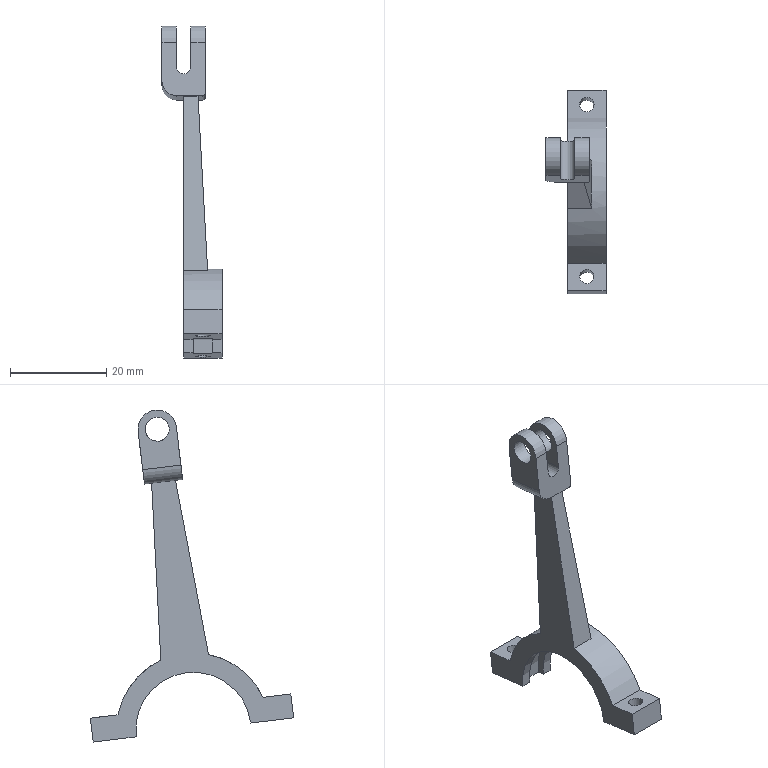Component | NX | 20A__27_2 | 1 solid | 33 faces | volume 3286 mm3 | plane 20 | cylinder 13 | commonest cylinder face diameters 3 x3 24 x2 5 x2 8 x2 32 x1 27 x1 1 x1 6 x1